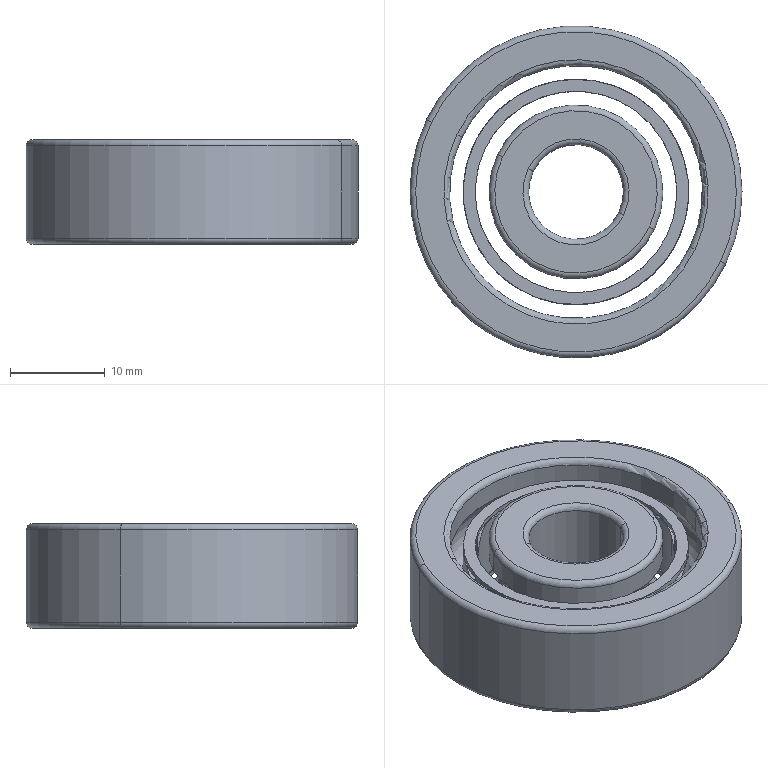Component | SolidWorks | DriveDevice-1_GB_T276-2013[DeepGrooveBallBearing[60000]6300]-1 | 12 solids | 119 faces | volume 6277 mm3 | cylinder 55 | plane 24 | torus 22 | sphere 18 | commonest cylinder face diameters 6.975 x19 23.75 x12 21.25 x12 26.667 x4 18.333 x4 35 x2 10 x2 | material AISI 304